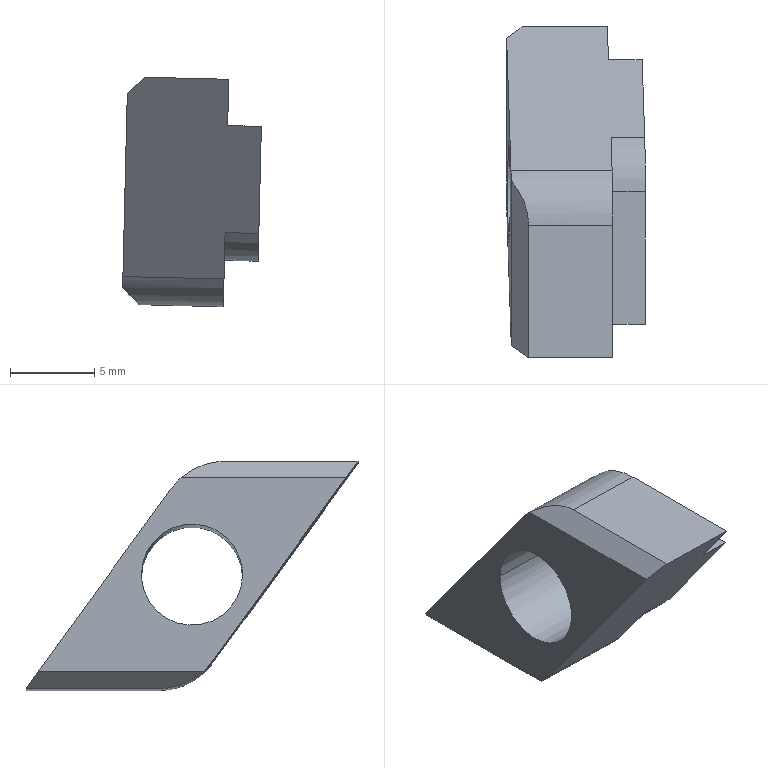Component | SolidWorks | 2012MB0201-1_AUpperRackFrameModule-1_ADJ42-G408-D6.5Assembly-10_RhombicNutAHG21-408-M6-1 | 1 solid | 18 faces | box 8.23 x 19.7 x 13.62 mm | volume 714 mm3 | plane 12 | cylinder 6 | commonest cylinder face diameters 8 x4 6 x2
STEP:
#1=CARTESIAN_POINT('',(-69.899,40.585,-44.875));
#2=VERTEX_POINT('',#1);
#3=CARTESIAN_POINT('',(-69.899,40.821,-44.875));
#4=VERTEX_POINT('',#3);
#5=CARTESIAN_POINT('',(-69.899,40.585,-44.875));
#6=CARTESIAN_POINT('',(-69.899,40.585,-44.89));
#7=CARTESIAN_POINT('',(-69.899,40.588,-44.905));
#8=CARTESIAN_POINT('',(-69.9,40.6,-44.934));
#9=CARTESIAN_POINT('',(-69.9,40.608,-44.947));
#10=CARTESIAN_POINT('',(-69.901,40.63,-44.969));
#11=CARTESIAN_POINT('',(-69.901,40.643,-44.978));
#12=CARTESIAN_POINT('',(-69.901,40.672,-44.99));
#13=CARTESIAN_POINT('',(-69.902,40.687,-44.993));
#14=CARTESIAN_POINT('',(-69.902,40.718,-44.993));
#15=CARTESIAN_POINT('',(-69.901,40.734,-44.99));
#16=CARTESIAN_POINT('',(-69.901,40.762,-44.978));
#17=CARTESIAN_POINT('',(-69.901,40.775,-44.969));
#18=CARTESIAN_POINT('',(-69.9,40.797,-44.947));
#19=CARTESIAN_POINT('',(-69.9,40.806,-44.934));
#20=CARTESIAN_POINT('',(-69.899,40.818,-44.905));
#21=CARTESIAN_POINT('',(-69.899,40.821,-44.89));
#22=CARTESIAN_POINT('',(-69.899,40.821,-44.875));
#23=B_SPLINE_CURVE_WITH_KNOTS('',3,(#5,#6,#7,#8,#9,#10,#11,#12,#13,#14,#15,#16,#17,#18,#19,#20,#21,#22),.UNSPECIFIED.,.F.,.F.,(4,2,2,2,2,2,2,2,4),(0.,0.0625,0.125,0.1875,0.25,0.3125,0.375,0.4375,0.5),.UNSPECIFIED.);
#24=EDGE_CURVE('',#2,#4,#23,.T.);
#25=ORIENTED_EDGE('',*,*,#24,.F.);
#26=CARTESIAN_POINT('',(-69.584,40.585,-44.882));
#27=VERTEX_POINT('',#26);
#28=CARTESIAN_POINT('',(-69.899,40.585,-44.875));
#29=DIRECTION('',(0.9997,0.,-0.02392));
#30=VECTOR('',#29,39.37);
#31=LINE('',#28,#30);
#32=EDGE_CURVE('',#2,#27,#31,.T.);
#33=ORIENTED_EDGE('',*,*,#32,.T.);
#34=CARTESIAN_POINT('',(-69.584,40.821,-44.882));
#35=VERTEX_POINT('',#34);
#36=CARTESIAN_POINT('',(-69.584,40.703,-44.882));
#37=DIRECTION('',(0.9997,0.,-0.02392));
#38=DIRECTION('',(0.,1.,0.));
#39=AXIS2_PLACEMENT_3D('',#36,#37,#38);
#40=CIRCLE('',#39,0.1181);
#41=EDGE_CURVE('',#27,#35,#40,.T.);
#42=ORIENTED_EDGE('',*,*,#41,.T.);
#43=CARTESIAN_POINT('',(-69.899,40.821,-44.875));
#44=DIRECTION('',(0.9997,0.,-0.02392));
#45=VECTOR('',#44,39.37);
#46=LINE('',#43,#45);
#47=EDGE_CURVE('',#4,#35,#46,.T.);
#48=ORIENTED_EDGE('',*,*,#47,.F.);
#49=EDGE_LOOP('',(#25,#33,#42,#48));
#50=FACE_OUTER_BOUND('',#49,.T.);
#51=CARTESIAN_POINT('',(-69.899,40.703,-44.875));
#52=DIRECTION('',(0.9997,0.,-0.02392));
#53=DIRECTION('',(0.,1.,0.));
#54=AXIS2_PLACEMENT_3D('',#51,#52,#53);
#55=CYLINDRICAL_SURFACE('',#54,0.1181);
#56=ADVANCED_FACE('',(#50),#55,.F.);
#57=CARTESIAN_POINT('',(-69.893,40.344,-44.648));
#58=VERTEX_POINT('',#57);
#59=CARTESIAN_POINT('',(-69.904,40.654,-45.075));
#60=VERTEX_POINT('',#59);
#61=CARTESIAN_POINT('',(-69.892,40.315,-44.609));
#62=DIRECTION('',(-0.01935,0.5878,-0.8088));
#63=VECTOR('',#62,39.37);
#64=LINE('',#61,#63);
#65=EDGE_CURVE('',#58,#60,#64,.T.);
#66=ORIENTED_EDGE('',*,*,#65,.F.);
#67=CARTESIAN_POINT('',(-69.893,40.728,-44.648));
#68=VERTEX_POINT('',#67);
#69=CARTESIAN_POINT('',(-69.893,40.303,-44.648));
#70=DIRECTION('',(-0.,1.,0.));
#71=VECTOR('',#70,39.37);
#72=LINE('',#69,#71);
#73=EDGE_CURVE('',#58,#68,#72,.T.);
#74=ORIENTED_EDGE('',*,*,#73,.T.);
#75=CARTESIAN_POINT('',(-69.894,40.752,-44.674));
#76=VERTEX_POINT('',#75);
#77=CARTESIAN_POINT('',(-69.896,40.624,-44.766));
#78=DIRECTION('',(0.9997,0.,-0.02392));
#79=DIRECTION('',(0.02392,0.,0.9997));
#80=AXIS2_PLACEMENT_3D('',#77,#78,#79);
#81=CIRCLE('',#80,0.1575);
#82=EDGE_CURVE('',#76,#68,#81,.T.);
#83=ORIENTED_EDGE('',*,*,#82,.F.);
#84=CARTESIAN_POINT('',(-69.904,41.062,-45.101));
#85=VERTEX_POINT('',#84);
#86=CARTESIAN_POINT('',(-69.905,41.091,-45.14));
#87=DIRECTION('',(0.01935,-0.5878,0.8088));
#88=VECTOR('',#87,39.37);
#89=LINE('',#86,#88);
#90=EDGE_CURVE('',#85,#76,#89,.T.);
#91=ORIENTED_EDGE('',*,*,#90,.F.);
#92=CARTESIAN_POINT('',(-69.904,40.677,-45.101));
#93=VERTEX_POINT('',#92);
#94=CARTESIAN_POINT('',(-69.904,40.303,-45.101));
#95=DIRECTION('',(-0.,1.,0.));
#96=VECTOR('',#95,39.37);
#97=LINE('',#94,#96);
#98=EDGE_CURVE('',#93,#85,#97,.T.);
#99=ORIENTED_EDGE('',*,*,#98,.F.);
#100=CARTESIAN_POINT('',(-69.901,40.781,-44.983));
#101=DIRECTION('',(0.9997,0.,-0.02392));
#102=DIRECTION('',(0.02392,0.,0.9997));
#103=AXIS2_PLACEMENT_3D('',#100,#101,#102);
#104=CIRCLE('',#103,0.1575);
#105=EDGE_CURVE('',#60,#93,#104,.T.);
#106=ORIENTED_EDGE('',*,*,#105,.F.);
#107=EDGE_LOOP('',(#66,#74,#83,#91,#99,#106));
#108=FACE_OUTER_BOUND('',#107,.T.);
#109=CARTESIAN_POINT('',(-69.899,40.821,-44.875));
#110=CARTESIAN_POINT('',(-69.898,40.821,-44.859));
#111=CARTESIAN_POINT('',(-69.898,40.818,-44.844));
#112=CARTESIAN_POINT('',(-69.897,40.806,-44.815));
#113=CARTESIAN_POINT('',(-69.897,40.797,-44.802));
#114=CARTESIAN_POINT('',(-69.896,40.775,-44.78));
#115=CARTESIAN_POINT('',(-69.896,40.762,-44.771));
#116=CARTESIAN_POINT('',(-69.896,40.734,-44.76));
#117=CARTESIAN_POINT('',(-69.896,40.718,-44.756));
#118=CARTESIAN_POINT('',(-69.896,40.687,-44.756));
#119=CARTESIAN_POINT('',(-69.896,40.672,-44.76));
#120=CARTESIAN_POINT('',(-69.896,40.643,-44.771));
#121=CARTESIAN_POINT('',(-69.896,40.63,-44.78));
#122=CARTESIAN_POINT('',(-69.897,40.608,-44.802));
#123=CARTESIAN_POINT('',(-69.897,40.6,-44.815));
#124=CARTESIAN_POINT('',(-69.898,40.588,-44.844));
#125=CARTESIAN_POINT('',(-69.898,40.585,-44.859));
#126=CARTESIAN_POINT('',(-69.899,40.585,-44.875));
#127=B_SPLINE_CURVE_WITH_KNOTS('',3,(#109,#110,#111,#112,#113,#114,#115,#116,#117,#118,#119,#120,#121,#122,#123,#124,#125,#126),.UNSPECIFIED.,.F.,.F.,(4,2,2,2,2,2,2,2,4),(0.5,0.5625,0.625,0.6875,0.75,0.8125,0.875,0.9375,1.),.UNSPECIFIED.);
#128=EDGE_CURVE('',#4,#2,#127,.T.);
#129=ORIENTED_EDGE('',*,*,#128,.T.);
#130=ORIENTED_EDGE('',*,*,#24,.T.);
#131=EDGE_LOOP('',(#129,#130));
#132=FACE_BOUND('',#131,.T.);
#133=CARTESIAN_POINT('',(-69.896,40.624,-44.766));
#134=DIRECTION('',(0.9997,0.,-0.02392));
#135=DIRECTION('',(0.02392,-0.,0.9997));
#136=AXIS2_PLACEMENT_3D('',#133,#134,#135);
#137=PLANE('',#136);
#138=ADVANCED_FACE('',(#108,#132),#137,.F.);
#139=CARTESIAN_POINT('',(-69.669,40.781,-45.146));
#140=VERTEX_POINT('',#139);
#141=CARTESIAN_POINT('',(-69.866,40.781,-45.141));
#142=VERTEX_POINT('',#141);
#143=CARTESIAN_POINT('',(-69.669,40.781,-45.146));
#144=DIRECTION('',(-0.9997,-0.,0.02392));
#145=VECTOR('',#144,39.37);
#146=LINE('',#143,#145);
#147=EDGE_CURVE('',#140,#142,#146,.T.);
#148=ORIENTED_EDGE('',*,*,#147,.T.);
#149=CARTESIAN_POINT('',(-69.866,41.091,-45.141));
#150=VERTEX_POINT('',#149);
#151=CARTESIAN_POINT('',(-69.866,40.303,-45.141));
#152=DIRECTION('',(-0.,1.,0.));
#153=VECTOR('',#152,39.37);
#154=LINE('',#151,#153);
#155=EDGE_CURVE('',#142,#150,#154,.T.);
#156=ORIENTED_EDGE('',*,*,#155,.T.);
#157=CARTESIAN_POINT('',(-69.669,41.091,-45.146));
#158=VERTEX_POINT('',#157);
#159=CARTESIAN_POINT('',(-69.669,41.091,-45.146));
#160=DIRECTION('',(-0.9997,-0.,0.02392));
#161=VECTOR('',#160,39.37);
#162=LINE('',#159,#161);
#163=EDGE_CURVE('',#158,#150,#162,.T.);
#164=ORIENTED_EDGE('',*,*,#163,.F.);
#165=CARTESIAN_POINT('',(-69.669,40.781,-45.146));
#166=DIRECTION('',(-0.,1.,0.));
#167=VECTOR('',#166,39.37);
#168=LINE('',#165,#167);
#169=EDGE_CURVE('',#140,#158,#168,.T.);
#170=ORIENTED_EDGE('',*,*,#169,.F.);
#171=EDGE_LOOP('',(#148,#156,#164,#170));
#172=FACE_OUTER_BOUND('',#171,.T.);
#173=CARTESIAN_POINT('',(-69.669,40.781,-45.146));
#174=DIRECTION('',(0.02392,-0.,0.9997));
#175=DIRECTION('',(0.9997,0.,-0.02392));
#176=AXIS2_PLACEMENT_3D('',#173,#174,#175);
#177=PLANE('',#176);
#178=ADVANCED_FACE('',(#172),#177,.F.);
#179=ORIENTED_EDGE('',*,*,#163,.T.);
#180=CARTESIAN_POINT('',(-69.79,41.147,-45.221));
#181=DIRECTION('',(-0.6137,-0.457,0.6438));
#182=VECTOR('',#181,39.37);
#183=LINE('',#180,#182);
#184=EDGE_CURVE('',#150,#85,#183,.T.);
#185=ORIENTED_EDGE('',*,*,#184,.T.);
#186=ORIENTED_EDGE('',*,*,#90,.T.);
#187=CARTESIAN_POINT('',(-69.658,40.752,-44.679));
#188=VERTEX_POINT('',#187);
#189=CARTESIAN_POINT('',(-69.658,40.752,-44.679));
#190=DIRECTION('',(-0.9997,-0.,0.02392));
#191=VECTOR('',#190,39.37);
#192=LINE('',#189,#191);
#193=EDGE_CURVE('',#188,#76,#192,.T.);
#194=ORIENTED_EDGE('',*,*,#193,.F.);
#195=CARTESIAN_POINT('',(-69.66,40.83,-44.788));
#196=VERTEX_POINT('',#195);
#197=CARTESIAN_POINT('',(-69.669,41.091,-45.146));
#198=DIRECTION('',(0.01935,-0.5878,0.8088));
#199=VECTOR('',#198,39.37);
#200=LINE('',#197,#199);
#201=EDGE_CURVE('',#196,#188,#200,.T.);
#202=ORIENTED_EDGE('',*,*,#201,.F.);
#203=CARTESIAN_POINT('',(-69.582,40.83,-44.79));
#204=VERTEX_POINT('',#203);
#205=CARTESIAN_POINT('',(-69.582,40.83,-44.79));
#206=DIRECTION('',(-0.9997,-0.,0.02392));
#207=VECTOR('',#206,39.37);
#208=LINE('',#205,#207);
#209=EDGE_CURVE('',#204,#196,#208,.T.);
#210=ORIENTED_EDGE('',*,*,#209,.F.);
#211=CARTESIAN_POINT('',(-69.588,41.012,-45.04));
#212=VERTEX_POINT('',#211);
#213=CARTESIAN_POINT('',(-69.588,41.012,-45.04));
#214=DIRECTION('',(0.01935,-0.5878,0.8088));
#215=VECTOR('',#214,39.37);
#216=LINE('',#213,#215);
#217=EDGE_CURVE('',#212,#204,#216,.T.);
#218=ORIENTED_EDGE('',*,*,#217,.F.);
#219=CARTESIAN_POINT('',(-69.666,41.012,-45.038));
#220=VERTEX_POINT('',#219);
#221=CARTESIAN_POINT('',(-69.588,41.012,-45.04));
#222=DIRECTION('',(-0.9997,-0.,0.02392));
#223=VECTOR('',#222,39.37);
#224=LINE('',#221,#223);
#225=EDGE_CURVE('',#212,#220,#224,.T.);
#226=ORIENTED_EDGE('',*,*,#225,.T.);
#227=CARTESIAN_POINT('',(-69.669,41.091,-45.146));
#228=DIRECTION('',(0.01935,-0.5878,0.8088));
#229=VECTOR('',#228,39.37);
#230=LINE('',#227,#229);
#231=EDGE_CURVE('',#158,#220,#230,.T.);
#232=ORIENTED_EDGE('',*,*,#231,.F.);
#233=EDGE_LOOP('',(#179,#185,#186,#194,#202,#210,#218,#226,#232));
#234=FACE_OUTER_BOUND('',#233,.T.);
#235=CARTESIAN_POINT('',(-69.669,41.091,-45.146));
#236=DIRECTION('',(-0.01406,-0.809,-0.5876));
#237=DIRECTION('',(-0.01935,0.5878,-0.8088));
#238=AXIS2_PLACEMENT_3D('',#235,#236,#237);
#239=PLANE('',#238);
#240=ADVANCED_FACE('',(#234),#239,.F.);
#241=ORIENTED_EDGE('',*,*,#155,.F.);
#242=CARTESIAN_POINT('',(-69.904,40.677,-45.101));
#243=CARTESIAN_POINT('',(-69.879,40.706,-45.127));
#244=CARTESIAN_POINT('',(-69.866,40.743,-45.141));
#245=CARTESIAN_POINT('',(-69.866,40.781,-45.141));
#246=(BOUNDED_CURVE()B_SPLINE_CURVE(3,(#242,#243,#244,#245),.UNSPECIFIED.,.F.,.F.)B_SPLINE_CURVE_WITH_KNOTS((4,4),(2.419,3.142),.UNSPECIFIED.)CURVE()GEOMETRIC_REPRESENTATION_ITEM()RATIONAL_B_SPLINE_CURVE((1.,0.9569,0.9569,1.))REPRESENTATION_ITEM(''));
#247=EDGE_CURVE('',#93,#142,#246,.T.);
#248=ORIENTED_EDGE('',*,*,#247,.F.);
#249=ORIENTED_EDGE('',*,*,#98,.T.);
#250=ORIENTED_EDGE('',*,*,#184,.F.);
#251=EDGE_LOOP('',(#241,#248,#249,#250));
#252=FACE_OUTER_BOUND('',#251,.T.);
#253=CARTESIAN_POINT('',(-69.904,40.303,-45.101));
#254=DIRECTION('',(0.7238,0.,0.69));
#255=DIRECTION('',(0.,-1.,-0.));
#256=AXIS2_PLACEMENT_3D('',#253,#254,#255);
#257=PLANE('',#256);
#258=ADVANCED_FACE('',(#252),#257,.F.);
#259=ORIENTED_EDGE('',*,*,#105,.T.);
#260=ORIENTED_EDGE('',*,*,#247,.T.);
#261=ORIENTED_EDGE('',*,*,#147,.F.);
#262=CARTESIAN_POINT('',(-69.667,40.654,-45.081));
#263=VERTEX_POINT('',#262);
#264=CARTESIAN_POINT('',(-69.665,40.781,-44.988));
#265=DIRECTION('',(0.9997,0.,-0.02392));
#266=DIRECTION('',(0.02392,0.,0.9997));
#267=AXIS2_PLACEMENT_3D('',#264,#265,#266);
#268=CIRCLE('',#267,0.1575);
#269=EDGE_CURVE('',#263,#140,#268,.T.);
#270=ORIENTED_EDGE('',*,*,#269,.F.);
#271=CARTESIAN_POINT('',(-69.667,40.654,-45.081));
#272=DIRECTION('',(-0.9997,-0.,0.02392));
#273=VECTOR('',#272,39.37);
#274=LINE('',#271,#273);
#275=EDGE_CURVE('',#263,#60,#274,.T.);
#276=ORIENTED_EDGE('',*,*,#275,.T.);
#277=EDGE_LOOP('',(#259,#260,#261,#270,#276));
#278=FACE_OUTER_BOUND('',#277,.T.);
#279=CARTESIAN_POINT('',(-69.665,40.781,-44.988));
#280=DIRECTION('',(0.9997,0.,-0.02392));
#281=DIRECTION('',(0.,-1.,0.));
#282=AXIS2_PLACEMENT_3D('',#279,#280,#281);
#283=CYLINDRICAL_SURFACE('',#282,0.1575);
#284=ADVANCED_FACE('',(#278),#283,.T.);
#285=ORIENTED_EDGE('',*,*,#82,.T.);
#286=CARTESIAN_POINT('',(-69.853,40.624,-44.61));
#287=VERTEX_POINT('',#286);
#288=CARTESIAN_POINT('',(-69.893,40.728,-44.648));
#289=CARTESIAN_POINT('',(-69.867,40.699,-44.623));
#290=CARTESIAN_POINT('',(-69.853,40.663,-44.61));
#291=CARTESIAN_POINT('',(-69.853,40.624,-44.61));
#292=(BOUNDED_CURVE()B_SPLINE_CURVE(3,(#288,#289,#290,#291),.UNSPECIFIED.,.F.,.F.)B_SPLINE_CURVE_WITH_KNOTS((4,4),(2.419,3.142),.UNSPECIFIED.)CURVE()GEOMETRIC_REPRESENTATION_ITEM()RATIONAL_B_SPLINE_CURVE((1.,0.9569,0.9569,1.))REPRESENTATION_ITEM(''));
#293=EDGE_CURVE('',#68,#287,#292,.T.);
#294=ORIENTED_EDGE('',*,*,#293,.T.);
#295=CARTESIAN_POINT('',(-69.656,40.624,-44.615));
#296=VERTEX_POINT('',#295);
#297=CARTESIAN_POINT('',(-69.656,40.624,-44.615));
#298=DIRECTION('',(-0.9997,-0.,0.02392));
#299=VECTOR('',#298,39.37);
#300=LINE('',#297,#299);
#301=EDGE_CURVE('',#296,#287,#300,.T.);
#302=ORIENTED_EDGE('',*,*,#301,.F.);
#303=CARTESIAN_POINT('',(-69.66,40.624,-44.772));
#304=DIRECTION('',(0.9997,0.,-0.02392));
#305=DIRECTION('',(0.02392,0.,0.9997));
#306=AXIS2_PLACEMENT_3D('',#303,#304,#305);
#307=CIRCLE('',#306,0.1575);
#308=EDGE_CURVE('',#188,#296,#307,.T.);
#309=ORIENTED_EDGE('',*,*,#308,.F.);
#310=ORIENTED_EDGE('',*,*,#193,.T.);
#311=EDGE_LOOP('',(#285,#294,#302,#309,#310));
#312=FACE_OUTER_BOUND('',#311,.T.);
#313=CARTESIAN_POINT('',(-69.66,40.624,-44.772));
#314=DIRECTION('',(0.9997,0.,-0.02392));
#315=DIRECTION('',(0.,-1.,0.));
#316=AXIS2_PLACEMENT_3D('',#313,#314,#315);
#317=CYLINDRICAL_SURFACE('',#316,0.1575);
#318=ADVANCED_FACE('',(#312),#317,.T.);
#319=CARTESIAN_POINT('',(-69.659,40.394,-44.723));
#320=VERTEX_POINT('',#319);
#321=CARTESIAN_POINT('',(-69.659,40.703,-44.723));
#322=VERTEX_POINT('',#321);
#323=CARTESIAN_POINT('',(-69.659,40.624,-44.723));
#324=DIRECTION('',(-0.,1.,0.));
#325=VECTOR('',#324,39.37);
#326=LINE('',#323,#325);
#327=EDGE_CURVE('',#320,#322,#326,.T.);
#328=ORIENTED_EDGE('',*,*,#327,.T.);
#329=CARTESIAN_POINT('',(-69.663,40.703,-44.88));
#330=DIRECTION('',(-0.9997,-0.,0.02392));
#331=DIRECTION('',(0.,1.,0.));
#332=AXIS2_PLACEMENT_3D('',#329,#330,#331);
#333=CIRCLE('',#332,0.1575);
#334=EDGE_CURVE('',#322,#196,#333,.T.);
#335=ORIENTED_EDGE('',*,*,#334,.T.);
#336=ORIENTED_EDGE('',*,*,#201,.T.);
#337=ORIENTED_EDGE('',*,*,#308,.T.);
#338=CARTESIAN_POINT('',(-69.656,40.315,-44.615));
#339=VERTEX_POINT('',#338);
#340=CARTESIAN_POINT('',(-69.656,40.624,-44.615));
#341=DIRECTION('',(0.,-1.,-0.));
#342=VECTOR('',#341,39.37);
#343=LINE('',#340,#342);
#344=EDGE_CURVE('',#296,#339,#343,.T.);
#345=ORIENTED_EDGE('',*,*,#344,.T.);
#346=CARTESIAN_POINT('',(-69.656,40.315,-44.615));
#347=DIRECTION('',(-0.01935,0.5878,-0.8088));
#348=VECTOR('',#347,39.37);
#349=LINE('',#346,#348);
#350=EDGE_CURVE('',#339,#320,#349,.T.);
#351=ORIENTED_EDGE('',*,*,#350,.T.);
#352=EDGE_LOOP('',(#328,#335,#336,#337,#345,#351));
#353=FACE_OUTER_BOUND('',#352,.T.);
#354=CARTESIAN_POINT('',(-69.66,40.624,-44.772));
#355=DIRECTION('',(0.9997,0.,-0.02392));
#356=DIRECTION('',(0.02392,-0.,0.9997));
#357=AXIS2_PLACEMENT_3D('',#354,#355,#356);
#358=PLANE('',#357);
#359=ADVANCED_FACE('',(#353),#358,.T.);
#360=ORIENTED_EDGE('',*,*,#334,.F.);
#361=CARTESIAN_POINT('',(-69.58,40.703,-44.725));
#362=VERTEX_POINT('',#361);
#363=CARTESIAN_POINT('',(-69.58,40.703,-44.725));
#364=DIRECTION('',(-0.9997,-0.,0.02392));
#365=VECTOR('',#364,39.37);
#366=LINE('',#363,#365);
#367=EDGE_CURVE('',#362,#322,#366,.T.);
#368=ORIENTED_EDGE('',*,*,#367,.F.);
#369=CARTESIAN_POINT('',(-69.584,40.703,-44.882));
#370=DIRECTION('',(0.9997,0.,-0.02392));
#371=DIRECTION('',(0.02392,0.,0.9997));
#372=AXIS2_PLACEMENT_3D('',#369,#370,#371);
#373=CIRCLE('',#372,0.1575);
#374=EDGE_CURVE('',#204,#362,#373,.T.);
#375=ORIENTED_EDGE('',*,*,#374,.F.);
#376=ORIENTED_EDGE('',*,*,#209,.T.);
#377=EDGE_LOOP('',(#360,#368,#375,#376));
#378=FACE_OUTER_BOUND('',#377,.T.);
#379=CARTESIAN_POINT('',(-69.584,40.703,-44.882));
#380=DIRECTION('',(0.9997,0.,-0.02392));
#381=DIRECTION('',(0.,-1.,0.));
#382=AXIS2_PLACEMENT_3D('',#379,#380,#381);
#383=CYLINDRICAL_SURFACE('',#382,0.1575);
#384=ADVANCED_FACE('',(#378),#383,.T.);
#385=CARTESIAN_POINT('',(-69.588,40.703,-45.04));
#386=VERTEX_POINT('',#385);
#387=CARTESIAN_POINT('',(-69.588,40.703,-45.04));
#388=DIRECTION('',(-0.,1.,0.));
#389=VECTOR('',#388,39.37);
#390=LINE('',#387,#389);
#391=EDGE_CURVE('',#386,#212,#390,.T.);
#392=ORIENTED_EDGE('',*,*,#391,.T.);
#393=ORIENTED_EDGE('',*,*,#217,.T.);
#394=ORIENTED_EDGE('',*,*,#374,.T.);
#395=CARTESIAN_POINT('',(-69.58,40.394,-44.725));
#396=VERTEX_POINT('',#395);
#397=CARTESIAN_POINT('',(-69.58,40.703,-44.725));
#398=DIRECTION('',(0.,-1.,-0.));
#399=VECTOR('',#398,39.37);
#400=LINE('',#397,#399);
#401=EDGE_CURVE('',#362,#396,#400,.T.);
#402=ORIENTED_EDGE('',*,*,#401,.T.);
#403=CARTESIAN_POINT('',(-69.586,40.575,-44.975));
#404=VERTEX_POINT('',#403);
#405=CARTESIAN_POINT('',(-69.58,40.394,-44.725));
#406=DIRECTION('',(-0.01935,0.5878,-0.8088));
#407=VECTOR('',#406,39.37);
#408=LINE('',#405,#407);
#409=EDGE_CURVE('',#396,#404,#408,.T.);
#410=ORIENTED_EDGE('',*,*,#409,.T.);
#411=CARTESIAN_POINT('',(-69.584,40.703,-44.882));
#412=DIRECTION('',(0.9997,0.,-0.02392));
#413=DIRECTION('',(0.02392,0.,0.9997));
#414=AXIS2_PLACEMENT_3D('',#411,#412,#413);
#415=CIRCLE('',#414,0.1575);
#416=EDGE_CURVE('',#404,#386,#415,.T.);
#417=ORIENTED_EDGE('',*,*,#416,.T.);
#418=EDGE_LOOP('',(#392,#393,#394,#402,#410,#417));
#419=FACE_OUTER_BOUND('',#418,.T.);
#420=CARTESIAN_POINT('',(-69.584,40.703,-44.882));
#421=DIRECTION('',(0.9997,0.,-0.02392));
#422=DIRECTION('',(0.,1.,0.));
#423=AXIS2_PLACEMENT_3D('',#420,#421,#422);
#424=CIRCLE('',#423,0.1181);
#425=EDGE_CURVE('',#35,#27,#424,.T.);
#426=ORIENTED_EDGE('',*,*,#425,.F.);
#427=ORIENTED_EDGE('',*,*,#41,.F.);
#428=EDGE_LOOP('',(#426,#427));
#429=FACE_BOUND('',#428,.T.);
#430=CARTESIAN_POINT('',(-69.584,40.703,-44.882));
#431=DIRECTION('',(0.9997,0.,-0.02392));
#432=DIRECTION('',(0.02392,-0.,0.9997));
#433=AXIS2_PLACEMENT_3D('',#430,#431,#432);
#434=PLANE('',#433);
#435=ADVANCED_FACE('',(#419,#429),#434,.T.);
#436=CARTESIAN_POINT('',(-69.666,40.703,-45.038));
#437=VERTEX_POINT('',#436);
#438=CARTESIAN_POINT('',(-69.666,40.624,-45.038));
#439=DIRECTION('',(0.,-1.,-0.));
#440=VECTOR('',#439,39.37);
#441=LINE('',#438,#440);
#442=EDGE_CURVE('',#220,#437,#441,.T.);
#443=ORIENTED_EDGE('',*,*,#442,.F.);
#444=ORIENTED_EDGE('',*,*,#225,.F.);
#445=ORIENTED_EDGE('',*,*,#391,.F.);
#446=CARTESIAN_POINT('',(-69.588,40.703,-45.04));
#447=DIRECTION('',(-0.9997,-0.,0.02392));
#448=VECTOR('',#447,39.37);
#449=LINE('',#446,#448);
#450=EDGE_CURVE('',#386,#437,#449,.T.);
#451=ORIENTED_EDGE('',*,*,#450,.T.);
#452=EDGE_LOOP('',(#443,#444,#445,#451));
#453=FACE_OUTER_BOUND('',#452,.T.);
#454=CARTESIAN_POINT('',(-69.588,40.703,-45.04));
#455=DIRECTION('',(0.02392,-0.,0.9997));
#456=DIRECTION('',(0.9997,0.,-0.02392));
#457=AXIS2_PLACEMENT_3D('',#454,#455,#456);
#458=PLANE('',#457);
#459=ADVANCED_FACE('',(#453),#458,.F.);
#460=ORIENTED_EDGE('',*,*,#231,.T.);
#461=ORIENTED_EDGE('',*,*,#442,.T.);
#462=CARTESIAN_POINT('',(-69.665,40.575,-44.973));
#463=VERTEX_POINT('',#462);
#464=CARTESIAN_POINT('',(-69.663,40.703,-44.88));
#465=DIRECTION('',(-0.9997,-0.,0.02392));
#466=DIRECTION('',(0.,1.,0.));
#467=AXIS2_PLACEMENT_3D('',#464,#465,#466);
#468=CIRCLE('',#467,0.1575);
#469=EDGE_CURVE('',#437,#463,#468,.T.);
#470=ORIENTED_EDGE('',*,*,#469,.T.);
#471=CARTESIAN_POINT('',(-69.656,40.315,-44.615));
#472=DIRECTION('',(-0.01935,0.5878,-0.8088));
#473=VECTOR('',#472,39.37);
#474=LINE('',#471,#473);
#475=EDGE_CURVE('',#463,#263,#474,.T.);
#476=ORIENTED_EDGE('',*,*,#475,.T.);
#477=ORIENTED_EDGE('',*,*,#269,.T.);
#478=ORIENTED_EDGE('',*,*,#169,.T.);
#479=EDGE_LOOP('',(#460,#461,#470,#476,#477,#478));
#480=FACE_OUTER_BOUND('',#479,.T.);
#481=CARTESIAN_POINT('',(-69.66,40.624,-44.772));
#482=DIRECTION('',(0.9997,0.,-0.02392));
#483=DIRECTION('',(0.02392,-0.,0.9997));
#484=AXIS2_PLACEMENT_3D('',#481,#482,#483);
#485=PLANE('',#484);
#486=ADVANCED_FACE('',(#480),#485,.T.);
#487=CARTESIAN_POINT('',(-69.853,40.315,-44.61));
#488=VERTEX_POINT('',#487);
#489=CARTESIAN_POINT('',(-69.656,40.315,-44.615));
#490=DIRECTION('',(-0.9997,-0.,0.02392));
#491=VECTOR('',#490,39.37);
#492=LINE('',#489,#491);
#493=EDGE_CURVE('',#339,#488,#492,.T.);
#494=ORIENTED_EDGE('',*,*,#493,.T.);
#495=CARTESIAN_POINT('',(-69.773,40.259,-44.534));
#496=DIRECTION('',(-0.6438,0.457,-0.6137));
#497=VECTOR('',#496,39.37);
#498=LINE('',#495,#497);
#499=EDGE_CURVE('',#488,#58,#498,.T.);
#500=ORIENTED_EDGE('',*,*,#499,.T.);
#501=ORIENTED_EDGE('',*,*,#65,.T.);
#502=ORIENTED_EDGE('',*,*,#275,.F.);
#503=ORIENTED_EDGE('',*,*,#475,.F.);
#504=CARTESIAN_POINT('',(-69.586,40.575,-44.975));
#505=DIRECTION('',(-0.9997,-0.,0.02392));
#506=VECTOR('',#505,39.37);
#507=LINE('',#504,#506);
#508=EDGE_CURVE('',#404,#463,#507,.T.);
#509=ORIENTED_EDGE('',*,*,#508,.F.);
#510=ORIENTED_EDGE('',*,*,#409,.F.);
#511=CARTESIAN_POINT('',(-69.58,40.394,-44.725));
#512=DIRECTION('',(-0.9997,-0.,0.02392));
#513=VECTOR('',#512,39.37);
#514=LINE('',#511,#513);
#515=EDGE_CURVE('',#396,#320,#514,.T.);
#516=ORIENTED_EDGE('',*,*,#515,.T.);
#517=ORIENTED_EDGE('',*,*,#350,.F.);
#518=EDGE_LOOP('',(#494,#500,#501,#502,#503,#509,#510,#516,#517));
#519=FACE_OUTER_BOUND('',#518,.T.);
#520=CARTESIAN_POINT('',(-69.656,40.315,-44.615));
#521=DIRECTION('',(0.01406,0.809,0.5876));
#522=DIRECTION('',(-0.9997,-0.,0.02392));
#523=AXIS2_PLACEMENT_3D('',#520,#521,#522);
#524=PLANE('',#523);
#525=ADVANCED_FACE('',(#519),#524,.F.);
#526=ORIENTED_EDGE('',*,*,#73,.F.);
#527=ORIENTED_EDGE('',*,*,#499,.F.);
#528=CARTESIAN_POINT('',(-69.853,40.303,-44.61));
#529=DIRECTION('',(-0.,1.,0.));
#530=VECTOR('',#529,39.37);
#531=LINE('',#528,#530);
#532=EDGE_CURVE('',#488,#287,#531,.T.);
#533=ORIENTED_EDGE('',*,*,#532,.T.);
#534=ORIENTED_EDGE('',*,*,#293,.F.);
#535=EDGE_LOOP('',(#526,#527,#533,#534));
#536=FACE_OUTER_BOUND('',#535,.T.);
#537=CARTESIAN_POINT('',(-69.853,40.303,-44.61));
#538=DIRECTION('',(0.69,0.,-0.7238));
#539=DIRECTION('',(-0.,1.,0.));
#540=AXIS2_PLACEMENT_3D('',#537,#538,#539);
#541=PLANE('',#540);
#542=ADVANCED_FACE('',(#536),#541,.F.);
#543=ORIENTED_EDGE('',*,*,#301,.T.);
#544=ORIENTED_EDGE('',*,*,#532,.F.);
#545=ORIENTED_EDGE('',*,*,#493,.F.);
#546=ORIENTED_EDGE('',*,*,#344,.F.);
#547=EDGE_LOOP('',(#543,#544,#545,#546));
#548=FACE_OUTER_BOUND('',#547,.T.);
#549=CARTESIAN_POINT('',(-69.656,40.624,-44.615));
#550=DIRECTION('',(-0.02392,0.,-0.9997));
#551=DIRECTION('',(-0.,1.,0.));
#552=AXIS2_PLACEMENT_3D('',#549,#550,#551);
#553=PLANE('',#552);
#554=ADVANCED_FACE('',(#548),#553,.F.);
#555=ORIENTED_EDGE('',*,*,#327,.F.);
#556=ORIENTED_EDGE('',*,*,#515,.F.);
#557=ORIENTED_EDGE('',*,*,#401,.F.);
#558=ORIENTED_EDGE('',*,*,#367,.T.);
#559=EDGE_LOOP('',(#555,#556,#557,#558));
#560=FACE_OUTER_BOUND('',#559,.T.);
#561=CARTESIAN_POINT('',(-69.58,40.703,-44.725));
#562=DIRECTION('',(-0.02392,0.,-0.9997));
#563=DIRECTION('',(-0.,1.,0.));
#564=AXIS2_PLACEMENT_3D('',#561,#562,#563);
#565=PLANE('',#564);
#566=ADVANCED_FACE('',(#560),#565,.F.);
#567=ORIENTED_EDGE('',*,*,#469,.F.);
#568=ORIENTED_EDGE('',*,*,#450,.F.);
#569=ORIENTED_EDGE('',*,*,#416,.F.);
#570=ORIENTED_EDGE('',*,*,#508,.T.);
#571=EDGE_LOOP('',(#567,#568,#569,#570));
#572=FACE_OUTER_BOUND('',#571,.T.);
#573=CARTESIAN_POINT('',(-69.584,40.703,-44.882));
#574=DIRECTION('',(0.9997,0.,-0.02392));
#575=DIRECTION('',(0.,-1.,0.));
#576=AXIS2_PLACEMENT_3D('',#573,#574,#575);
#577=CYLINDRICAL_SURFACE('',#576,0.1575);
#578=ADVANCED_FACE('',(#572),#577,.T.);
#579=ORIENTED_EDGE('',*,*,#32,.F.);
#580=ORIENTED_EDGE('',*,*,#128,.F.);
#581=ORIENTED_EDGE('',*,*,#47,.T.);
#582=ORIENTED_EDGE('',*,*,#425,.T.);
#583=EDGE_LOOP('',(#579,#580,#581,#582));
#584=FACE_OUTER_BOUND('',#583,.T.);
#585=CARTESIAN_POINT('',(-69.899,40.703,-44.875));
#586=DIRECTION('',(0.9997,0.,-0.02392));
#587=DIRECTION('',(0.,1.,0.));
#588=AXIS2_PLACEMENT_3D('',#585,#586,#587);
#589=CYLINDRICAL_SURFACE('',#588,0.1181);
#590=ADVANCED_FACE('',(#584),#589,.F.);
#591=CLOSED_SHELL('',(#56,#138,#178,#240,#258,#284,#318,#359,#384,#435,#459,#486,#525,#542,#554,#566,#578,#590));
#592=MANIFOLD_SOLID_BREP('',#591);
#593=CARTESIAN_POINT('',(0.,0.,0.));
#594=DIRECTION('',(0.,0.,1.));
#595=DIRECTION('',(1.,0.,0.));
#596=AXIS2_PLACEMENT_3D('',#593,#594,#595);
#597=(LENGTH_UNIT()NAMED_UNIT(*)SI_UNIT($,.METRE.));
#598=LENGTH_MEASURE_WITH_UNIT(LENGTH_MEASURE(0.0254),#597);
#599=DIMENSIONAL_EXPONENTS(1.,0.,0.,0.,0.,0.,0.);
#600=(CONVERSION_BASED_UNIT('',#598)LENGTH_UNIT()NAMED_UNIT(#599));
#601=UNCERTAINTY_MEASURE_WITH_UNIT(LENGTH_MEASURE(0.00001),#600,'','');
#602=(NAMED_UNIT(*)PLANE_ANGLE_UNIT()SI_UNIT($,.RADIAN.));
#603=(NAMED_UNIT(*)SI_UNIT($,.STERADIAN.)SOLID_ANGLE_UNIT());
#604=(GEOMETRIC_REPRESENTATION_CONTEXT(3)GLOBAL_UNCERTAINTY_ASSIGNED_CONTEXT((#601))GLOBAL_UNIT_ASSIGNED_CONTEXT((#600,#602,#603))REPRESENTATION_CONTEXT('',''));
#605=ADVANCED_BREP_SHAPE_REPRESENTATION('',(#592,#596),#604);
#606=COLOUR_RGB('',0.7922,0.8196,0.9333);
#607=FILL_AREA_STYLE_COLOUR('',#606);
#608=FILL_AREA_STYLE('',(#607));
#609=SURFACE_STYLE_FILL_AREA(#608);
#610=SURFACE_SIDE_STYLE('',(#609));
#611=SURFACE_STYLE_USAGE(.BOTH.,#610);
#612=PRESENTATION_STYLE_ASSIGNMENT((#611));
#613=STYLED_ITEM('',(#612),#592);
#614=PRESENTATION_LAYER_ASSIGNMENT('','',(#613));
#615=(LENGTH_UNIT()NAMED_UNIT(*)SI_UNIT($,.METRE.));
#616=LENGTH_MEASURE_WITH_UNIT(LENGTH_MEASURE(0.0254),#615);
#617=DIMENSIONAL_EXPONENTS(1.,0.,0.,0.,0.,0.,0.);
#618=(CONVERSION_BASED_UNIT('',#616)LENGTH_UNIT()NAMED_UNIT(#617));
#619=UNCERTAINTY_MEASURE_WITH_UNIT(LENGTH_MEASURE(0.00001),#618,'','');
#620=(NAMED_UNIT(*)PLANE_ANGLE_UNIT()SI_UNIT($,.RADIAN.));
#621=(NAMED_UNIT(*)SI_UNIT($,.STERADIAN.)SOLID_ANGLE_UNIT());
#622=(GEOMETRIC_REPRESENTATION_CONTEXT(3)GLOBAL_UNCERTAINTY_ASSIGNED_CONTEXT((#619))GLOBAL_UNIT_ASSIGNED_CONTEXT((#618,#620,#621))REPRESENTATION_CONTEXT('',''));
#623=MECHANICAL_DESIGN_GEOMETRIC_PRESENTATION_REPRESENTATION('',(#613),#622);